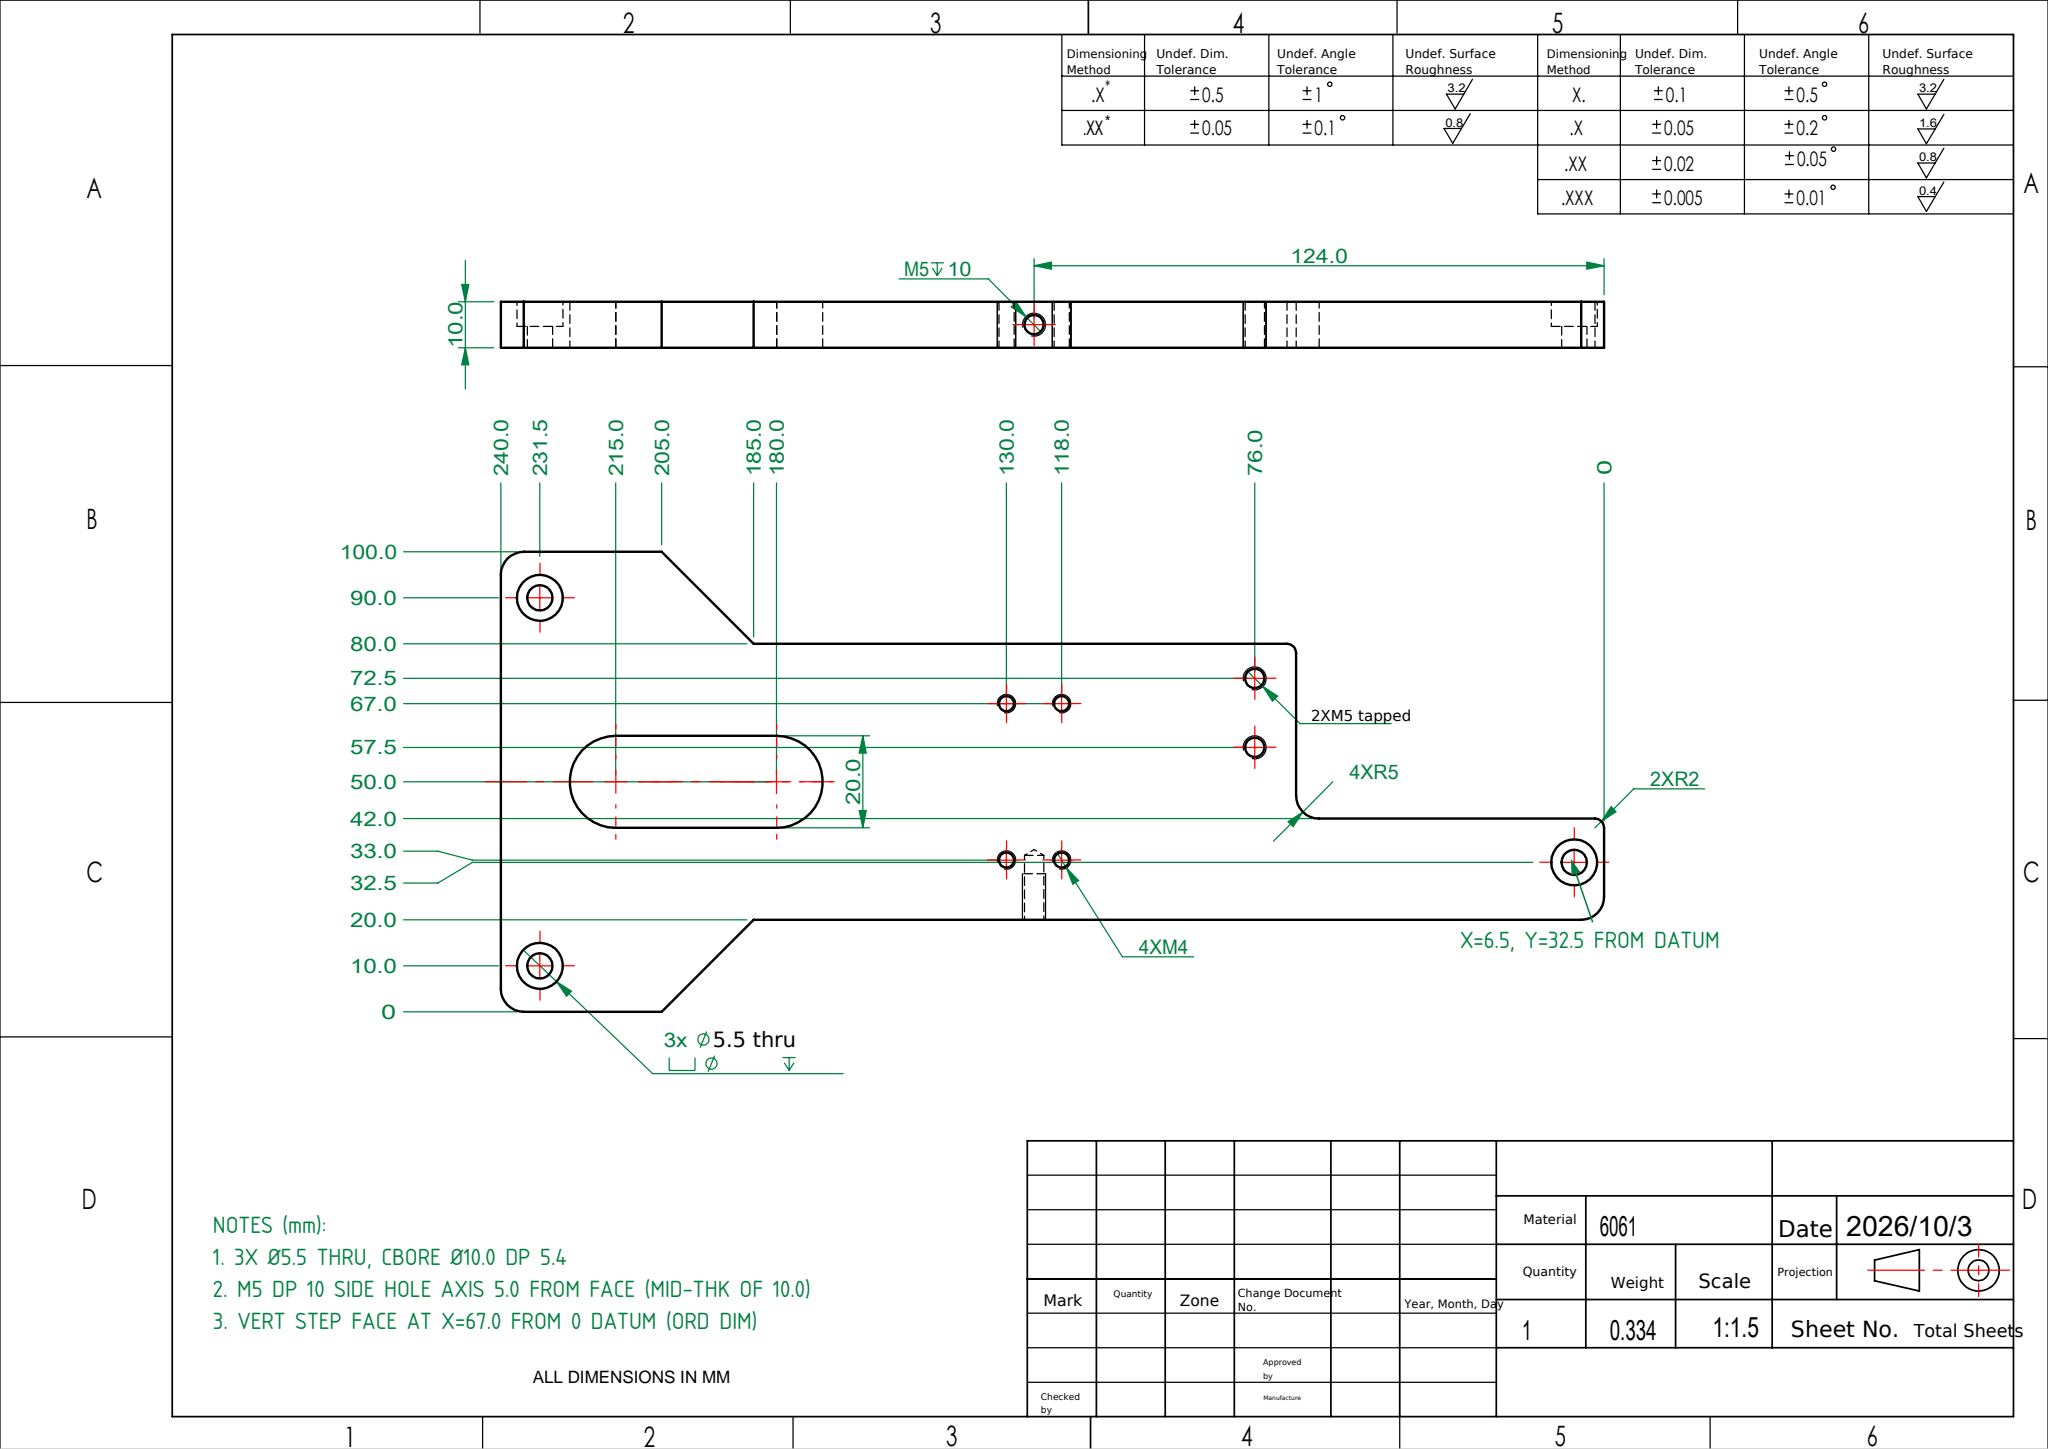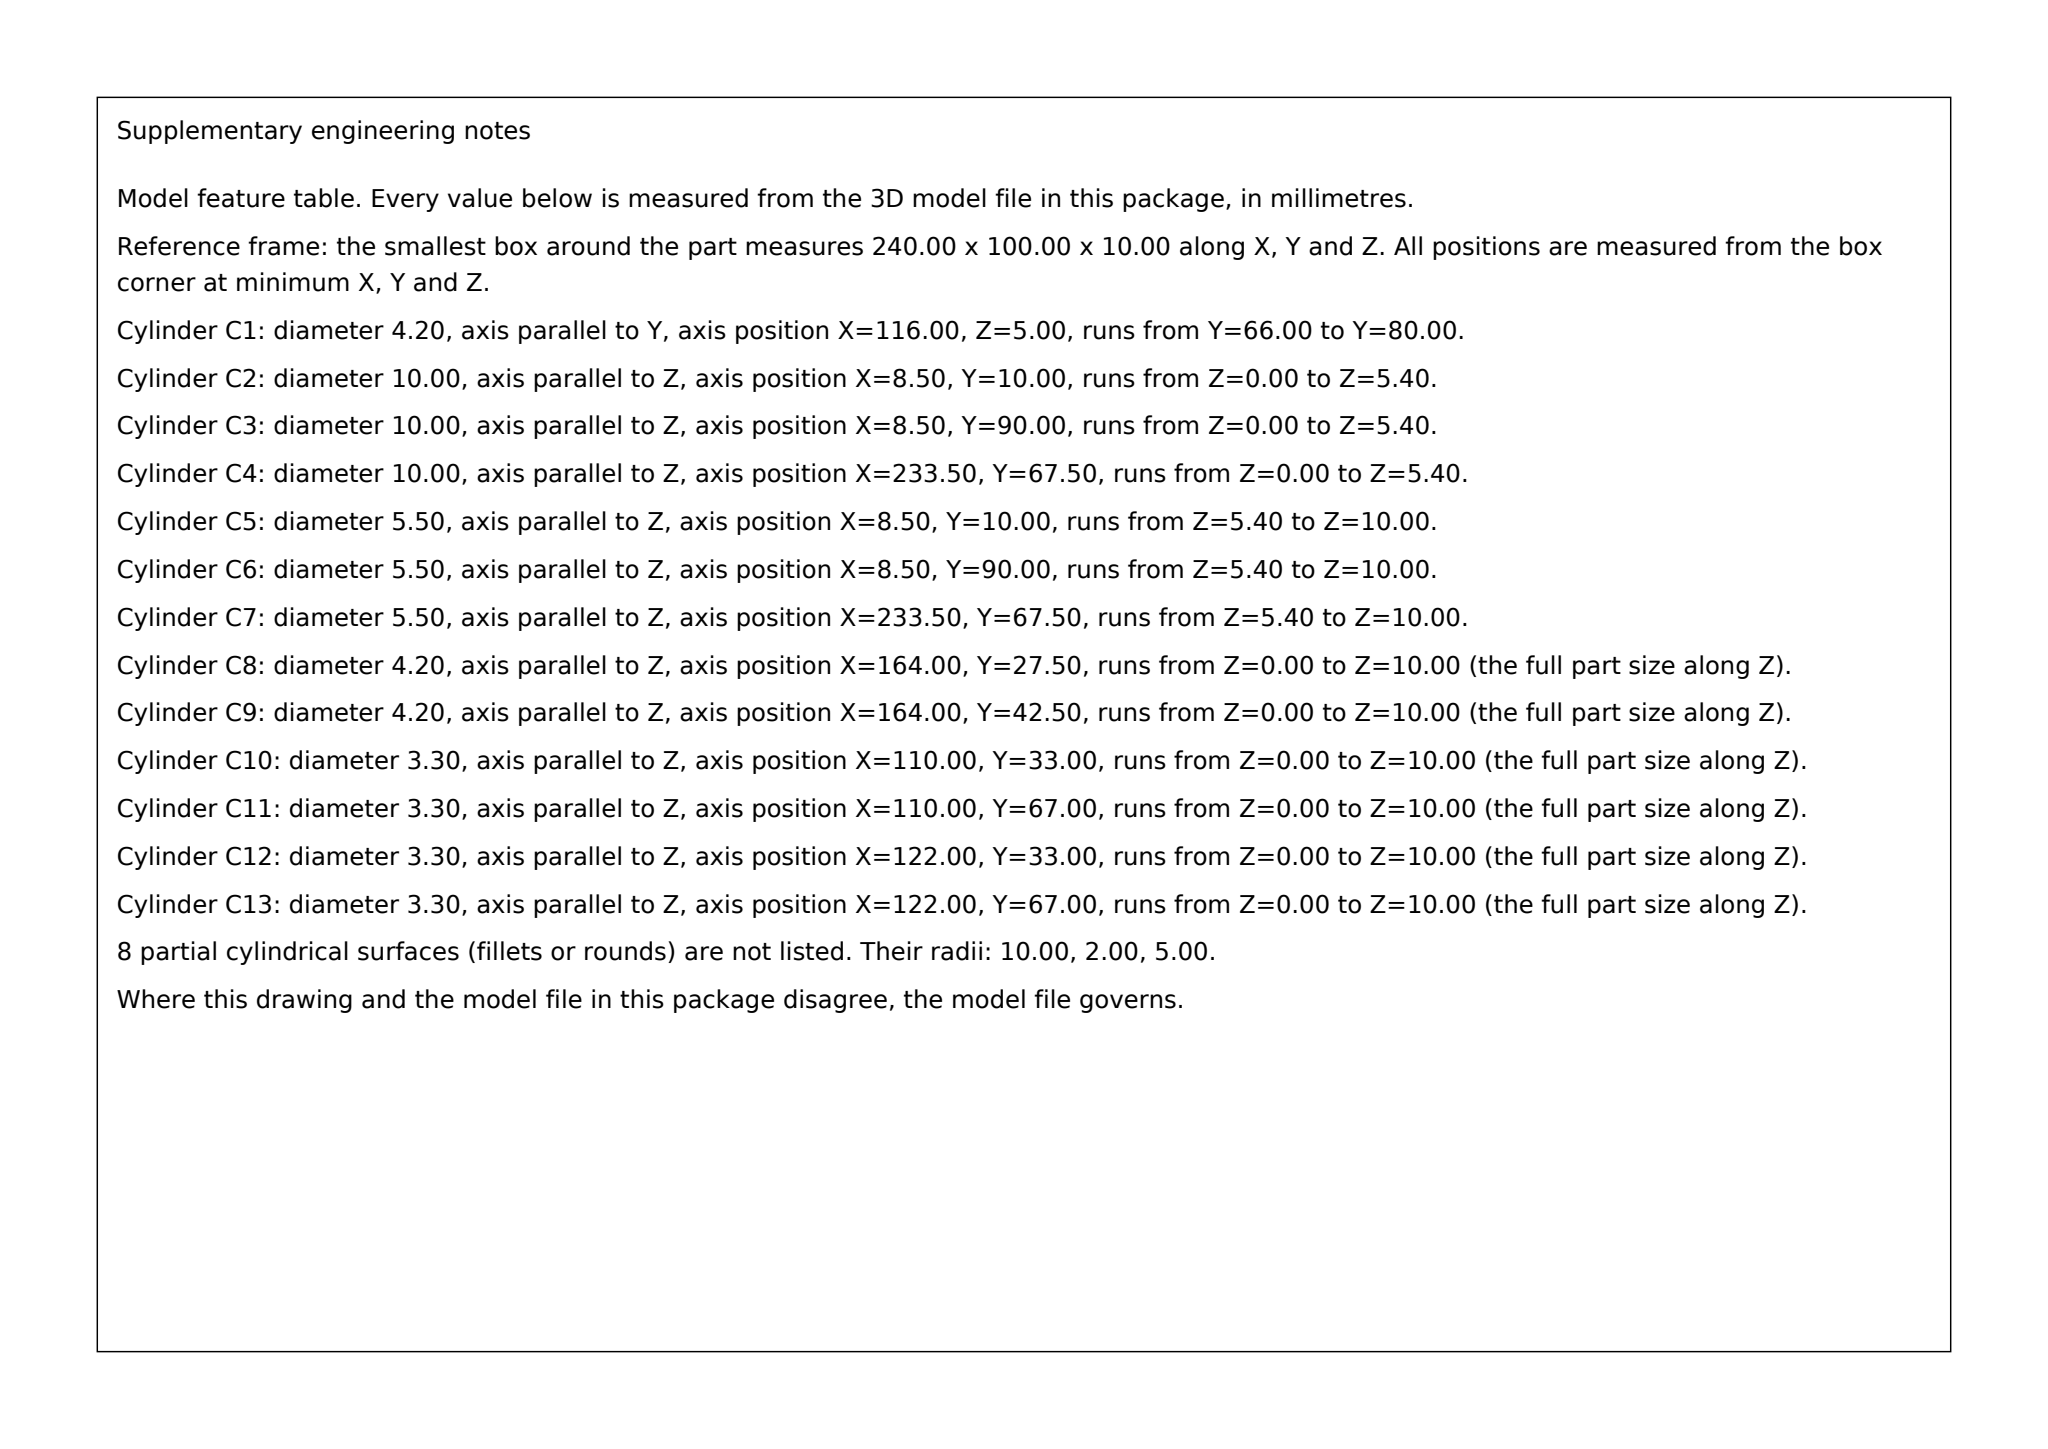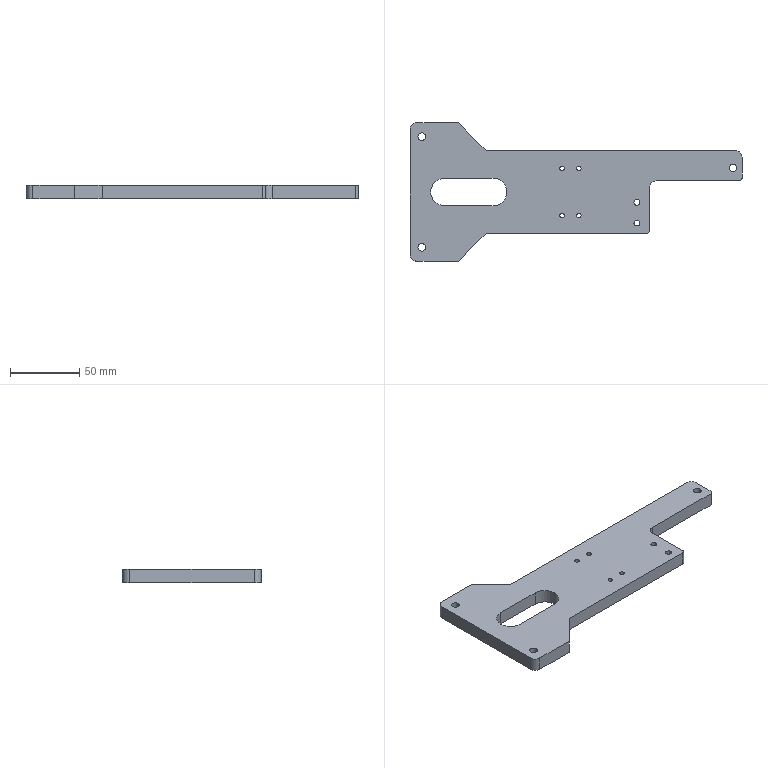Part | SolidWorks | mm | material 6061 | 1 solid | 54 faces | box 240 x 100 x 10 mm | volume 123855 mm3 | cylinder 35 | plane 17 | cone 2 | commonest cylinder face diameters 10 x10 3.3 x8 4.2 x6 5.5 x6 20 x3 4 x2
Drawing notes:
3X Ø5.5 THRU, CBORE Ø10.0 DP 5.4 | from the solid: Ø10 c'bore cylinders length 5.4 (z-planes at 5.4) over Ø5.5 thru holes
3RD Ø5.5/CBORE Ø10 HOLE AT X=6.5 FROM 0 DATUM, Y=32.5 | from the solid: Ø5.5/Ø10 c'bore at x=233.5 from bbox min = 240-233.5 = 6.5 from 0 datum edge; y=67.5 -> 32.5
M5 DP 10 SIDE HOLE AXIS 5.0 FROM FACE (MID-THK OF 10.0) | from the solid: Ø4.2 y-axis hole at z=5.0, plate z-planes 0 to 10.0
VERT STEP FACE AT X=67.0 FROM 0 DATUM (ORD DIM) | from the solid: axis_plane x=173.0 of bbox 240 wide; 240-173=67.0 from drawing 0 datum at right edge